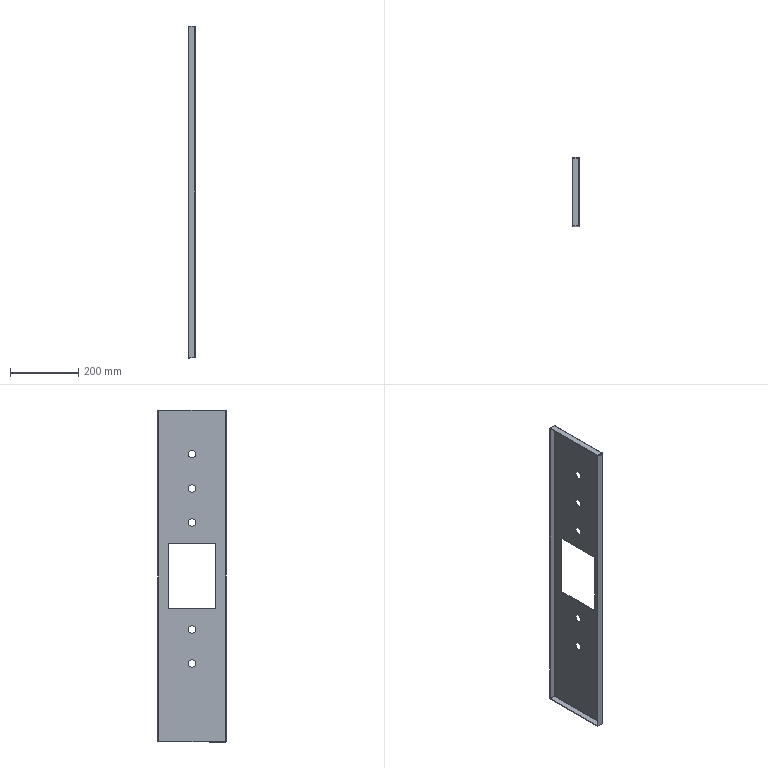Component | SolidWorks | 30-01A-1_TouchScreenPanel-1 | 1 solid | 52 faces | volume 411152 mm3 | plane 26 | cylinder 18 | spline 8 | commonest cylinder face diameters 22 x10 5.473 x4 1.473 x4